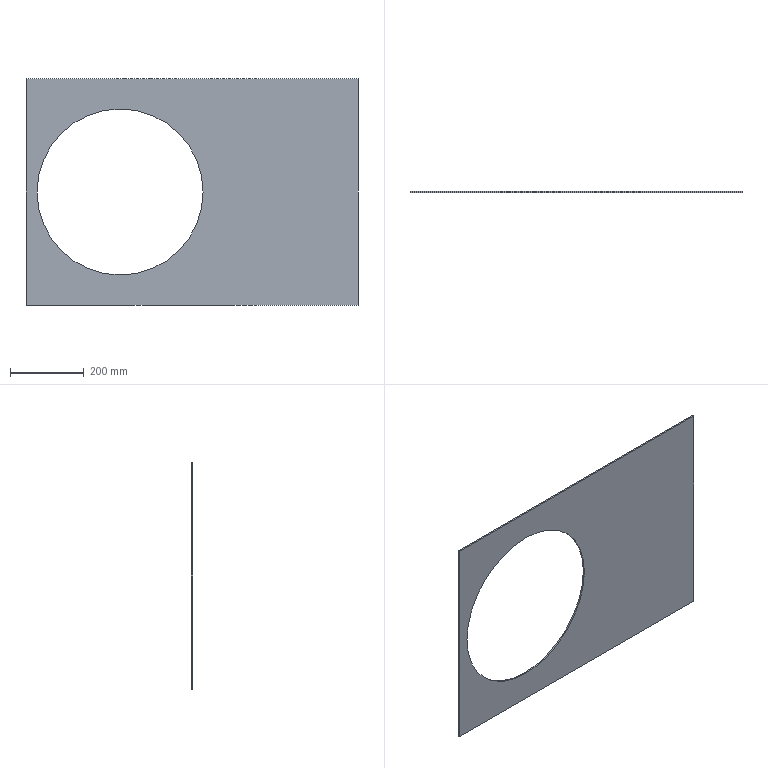Component | SolidWorks | Panel-1 | 1 solid | 8 faces | box 900 x 4 x 615 mm | volume 1577827 mm3 | plane 6 | cylinder 2 | commonest cylinder face diameters 450 x2
build123d program:
from build123d import *

# Parameters (mm, degrees)
SKETCH1_W      = 900
SKETCH1_H      = 615
SKETCH1_R      = 225
EXTRUDE1_DEPTH = 4


with BuildPart() as part:
    # Sketch1 → Extrude1 (new body)
    with BuildSketch(Plane(origin=(0, 0, 0), x_dir=(1, 0, 0), z_dir=(0, 1, 0))):
        with Locations((392.086, -275.962)):
            Rectangle(SKETCH1_W, SKETCH1_H)
        with Locations(Location((197.086, -275.962, 0), (0, 0, 270))):
            Circle(SKETCH1_R, mode=Mode.SUBTRACT)
    extrude(amount=EXTRUDE1_DEPTH)


solid = part.part

# Placed as in the assembly
solid = solid.moved(Location((-361.87, 366.983, -271.962), (0, 0, 0)))
STEP:
#1=CARTESIAN_POINT('',(-6.488,14.606,-8.701));
#2=VERTEX_POINT('',#1);
#3=CARTESIAN_POINT('',(-6.488,14.606,9.016));
#4=VERTEX_POINT('',#3);
#5=CARTESIAN_POINT('',(-6.488,14.606,0.1575));
#6=DIRECTION('',(0.,1.,0.));
#7=DIRECTION('',(0.,0.,1.));
#8=AXIS2_PLACEMENT_3D('',#5,#6,#7);
#9=CIRCLE('',#8,8.858);
#10=EDGE_CURVE('',#2,#4,#9,.T.);
#11=ORIENTED_EDGE('',*,*,#10,.T.);
#12=CARTESIAN_POINT('',(-6.488,14.448,9.016));
#13=VERTEX_POINT('',#12);
#14=CARTESIAN_POINT('',(-6.488,14.606,9.016));
#15=DIRECTION('',(0.,-1.,0.));
#16=VECTOR('',#15,39.37);
#17=LINE('',#14,#16);
#18=EDGE_CURVE('',#4,#13,#17,.T.);
#19=ORIENTED_EDGE('',*,*,#18,.T.);
#20=CARTESIAN_POINT('',(-6.488,14.448,-8.701));
#21=VERTEX_POINT('',#20);
#22=CARTESIAN_POINT('',(-6.488,14.448,0.1575));
#23=DIRECTION('',(0.,1.,0.));
#24=DIRECTION('',(0.,0.,1.));
#25=AXIS2_PLACEMENT_3D('',#22,#23,#24);
#26=CIRCLE('',#25,8.858);
#27=EDGE_CURVE('',#21,#13,#26,.T.);
#28=ORIENTED_EDGE('',*,*,#27,.F.);
#29=CARTESIAN_POINT('',(-6.488,14.606,-8.701));
#30=DIRECTION('',(0.,-1.,0.));
#31=VECTOR('',#30,39.37);
#32=LINE('',#29,#31);
#33=EDGE_CURVE('',#2,#21,#32,.T.);
#34=ORIENTED_EDGE('',*,*,#33,.F.);
#35=EDGE_LOOP('',(#11,#19,#28,#34));
#36=FACE_OUTER_BOUND('',#35,.T.);
#37=CARTESIAN_POINT('',(-6.488,14.606,0.1575));
#38=DIRECTION('',(0.,-1.,0.));
#39=DIRECTION('',(0.,0.,-1.));
#40=AXIS2_PLACEMENT_3D('',#37,#38,#39);
#41=CYLINDRICAL_SURFACE('',#40,8.858);
#42=ADVANCED_FACE('',(#36),#41,.F.);
#43=CARTESIAN_POINT('',(-16.527,14.606,-11.949));
#44=VERTEX_POINT('',#43);
#45=CARTESIAN_POINT('',(-16.527,14.606,12.264));
#46=VERTEX_POINT('',#45);
#47=CARTESIAN_POINT('',(-16.527,14.606,-11.949));
#48=DIRECTION('',(-0.,0.,1.));
#49=VECTOR('',#48,39.37);
#50=LINE('',#47,#49);
#51=EDGE_CURVE('',#44,#46,#50,.T.);
#52=ORIENTED_EDGE('',*,*,#51,.T.);
#53=CARTESIAN_POINT('',(18.906,14.606,12.264));
#54=VERTEX_POINT('',#53);
#55=CARTESIAN_POINT('',(-16.527,14.606,12.264));
#56=DIRECTION('',(1.,0.,0.));
#57=VECTOR('',#56,39.37);
#58=LINE('',#55,#57);
#59=EDGE_CURVE('',#46,#54,#58,.T.);
#60=ORIENTED_EDGE('',*,*,#59,.T.);
#61=CARTESIAN_POINT('',(18.906,14.606,-11.949));
#62=VERTEX_POINT('',#61);
#63=CARTESIAN_POINT('',(18.906,14.606,-11.949));
#64=DIRECTION('',(-0.,0.,-1.));
#65=VECTOR('',#64,39.37);
#66=LINE('',#63,#65);
#67=EDGE_CURVE('',#54,#62,#66,.T.);
#68=ORIENTED_EDGE('',*,*,#67,.T.);
#69=CARTESIAN_POINT('',(-16.527,14.606,-11.949));
#70=DIRECTION('',(-1.,0.,-0.));
#71=VECTOR('',#70,39.37);
#72=LINE('',#69,#71);
#73=EDGE_CURVE('',#62,#44,#72,.T.);
#74=ORIENTED_EDGE('',*,*,#73,.T.);
#75=EDGE_LOOP('',(#52,#60,#68,#74));
#76=FACE_OUTER_BOUND('',#75,.T.);
#77=ORIENTED_EDGE('',*,*,#10,.F.);
#78=CARTESIAN_POINT('',(-6.488,14.606,0.1575));
#79=DIRECTION('',(0.,1.,0.));
#80=DIRECTION('',(0.,0.,1.));
#81=AXIS2_PLACEMENT_3D('',#78,#79,#80);
#82=CIRCLE('',#81,8.858);
#83=EDGE_CURVE('',#4,#2,#82,.T.);
#84=ORIENTED_EDGE('',*,*,#83,.F.);
#85=EDGE_LOOP('',(#77,#84));
#86=FACE_BOUND('',#85,.T.);
#87=CARTESIAN_POINT('',(-16.527,14.606,12.264));
#88=DIRECTION('',(0.,1.,0.));
#89=DIRECTION('',(0.,0.,1.));
#90=AXIS2_PLACEMENT_3D('',#87,#88,#89);
#91=PLANE('',#90);
#92=ADVANCED_FACE('',(#76,#86),#91,.T.);
#93=CARTESIAN_POINT('',(-16.527,14.448,-11.949));
#94=VERTEX_POINT('',#93);
#95=CARTESIAN_POINT('',(-16.527,14.448,12.264));
#96=VERTEX_POINT('',#95);
#97=CARTESIAN_POINT('',(-16.527,14.448,-11.949));
#98=DIRECTION('',(-0.,0.,1.));
#99=VECTOR('',#98,39.37);
#100=LINE('',#97,#99);
#101=EDGE_CURVE('',#94,#96,#100,.T.);
#102=ORIENTED_EDGE('',*,*,#101,.F.);
#103=CARTESIAN_POINT('',(18.906,14.448,-11.949));
#104=VERTEX_POINT('',#103);
#105=CARTESIAN_POINT('',(-16.527,14.448,-11.949));
#106=DIRECTION('',(-1.,0.,-0.));
#107=VECTOR('',#106,39.37);
#108=LINE('',#105,#107);
#109=EDGE_CURVE('',#104,#94,#108,.T.);
#110=ORIENTED_EDGE('',*,*,#109,.F.);
#111=CARTESIAN_POINT('',(18.906,14.448,12.264));
#112=VERTEX_POINT('',#111);
#113=CARTESIAN_POINT('',(18.906,14.448,-11.949));
#114=DIRECTION('',(-0.,0.,-1.));
#115=VECTOR('',#114,39.37);
#116=LINE('',#113,#115);
#117=EDGE_CURVE('',#112,#104,#116,.T.);
#118=ORIENTED_EDGE('',*,*,#117,.F.);
#119=CARTESIAN_POINT('',(-16.527,14.448,12.264));
#120=DIRECTION('',(1.,0.,0.));
#121=VECTOR('',#120,39.37);
#122=LINE('',#119,#121);
#123=EDGE_CURVE('',#96,#112,#122,.T.);
#124=ORIENTED_EDGE('',*,*,#123,.F.);
#125=EDGE_LOOP('',(#102,#110,#118,#124));
#126=FACE_OUTER_BOUND('',#125,.T.);
#127=ORIENTED_EDGE('',*,*,#27,.T.);
#128=CARTESIAN_POINT('',(-6.488,14.448,0.1575));
#129=DIRECTION('',(0.,1.,0.));
#130=DIRECTION('',(0.,0.,1.));
#131=AXIS2_PLACEMENT_3D('',#128,#129,#130);
#132=CIRCLE('',#131,8.858);
#133=EDGE_CURVE('',#13,#21,#132,.T.);
#134=ORIENTED_EDGE('',*,*,#133,.T.);
#135=EDGE_LOOP('',(#127,#134));
#136=FACE_BOUND('',#135,.T.);
#137=CARTESIAN_POINT('',(-16.527,14.448,12.264));
#138=DIRECTION('',(0.,1.,0.));
#139=DIRECTION('',(0.,0.,1.));
#140=AXIS2_PLACEMENT_3D('',#137,#138,#139);
#141=PLANE('',#140);
#142=ADVANCED_FACE('',(#126,#136),#141,.F.);
#143=ORIENTED_EDGE('',*,*,#101,.T.);
#144=CARTESIAN_POINT('',(-16.527,14.606,12.264));
#145=DIRECTION('',(0.,-1.,0.));
#146=VECTOR('',#145,39.37);
#147=LINE('',#144,#146);
#148=EDGE_CURVE('',#46,#96,#147,.T.);
#149=ORIENTED_EDGE('',*,*,#148,.F.);
#150=ORIENTED_EDGE('',*,*,#51,.F.);
#151=CARTESIAN_POINT('',(-16.527,14.606,-11.949));
#152=DIRECTION('',(0.,-1.,0.));
#153=VECTOR('',#152,39.37);
#154=LINE('',#151,#153);
#155=EDGE_CURVE('',#44,#94,#154,.T.);
#156=ORIENTED_EDGE('',*,*,#155,.T.);
#157=EDGE_LOOP('',(#143,#149,#150,#156));
#158=FACE_OUTER_BOUND('',#157,.T.);
#159=CARTESIAN_POINT('',(-16.527,14.606,-11.949));
#160=DIRECTION('',(1.,0.,0.));
#161=DIRECTION('',(0.,0.,-1.));
#162=AXIS2_PLACEMENT_3D('',#159,#160,#161);
#163=PLANE('',#162);
#164=ADVANCED_FACE('',(#158),#163,.F.);
#165=ORIENTED_EDGE('',*,*,#123,.T.);
#166=CARTESIAN_POINT('',(18.906,14.606,12.264));
#167=DIRECTION('',(0.,-1.,0.));
#168=VECTOR('',#167,39.37);
#169=LINE('',#166,#168);
#170=EDGE_CURVE('',#54,#112,#169,.T.);
#171=ORIENTED_EDGE('',*,*,#170,.F.);
#172=ORIENTED_EDGE('',*,*,#59,.F.);
#173=ORIENTED_EDGE('',*,*,#148,.T.);
#174=EDGE_LOOP('',(#165,#171,#172,#173));
#175=FACE_OUTER_BOUND('',#174,.T.);
#176=CARTESIAN_POINT('',(-16.527,14.606,12.264));
#177=DIRECTION('',(0.,0.,-1.));
#178=DIRECTION('',(-1.,0.,0.));
#179=AXIS2_PLACEMENT_3D('',#176,#177,#178);
#180=PLANE('',#179);
#181=ADVANCED_FACE('',(#175),#180,.F.);
#182=ORIENTED_EDGE('',*,*,#117,.T.);
#183=CARTESIAN_POINT('',(18.906,14.606,-11.949));
#184=DIRECTION('',(0.,-1.,0.));
#185=VECTOR('',#184,39.37);
#186=LINE('',#183,#185);
#187=EDGE_CURVE('',#62,#104,#186,.T.);
#188=ORIENTED_EDGE('',*,*,#187,.F.);
#189=ORIENTED_EDGE('',*,*,#67,.F.);
#190=ORIENTED_EDGE('',*,*,#170,.T.);
#191=EDGE_LOOP('',(#182,#188,#189,#190));
#192=FACE_OUTER_BOUND('',#191,.T.);
#193=CARTESIAN_POINT('',(18.906,14.606,-11.949));
#194=DIRECTION('',(-1.,0.,0.));
#195=DIRECTION('',(0.,0.,1.));
#196=AXIS2_PLACEMENT_3D('',#193,#194,#195);
#197=PLANE('',#196);
#198=ADVANCED_FACE('',(#192),#197,.F.);
#199=ORIENTED_EDGE('',*,*,#109,.T.);
#200=ORIENTED_EDGE('',*,*,#155,.F.);
#201=ORIENTED_EDGE('',*,*,#73,.F.);
#202=ORIENTED_EDGE('',*,*,#187,.T.);
#203=EDGE_LOOP('',(#199,#200,#201,#202));
#204=FACE_OUTER_BOUND('',#203,.T.);
#205=CARTESIAN_POINT('',(-16.527,14.606,-11.949));
#206=DIRECTION('',(-0.,0.,1.));
#207=DIRECTION('',(1.,0.,0.));
#208=AXIS2_PLACEMENT_3D('',#205,#206,#207);
#209=PLANE('',#208);
#210=ADVANCED_FACE('',(#204),#209,.F.);
#211=ORIENTED_EDGE('',*,*,#18,.F.);
#212=ORIENTED_EDGE('',*,*,#83,.T.);
#213=ORIENTED_EDGE('',*,*,#33,.T.);
#214=ORIENTED_EDGE('',*,*,#133,.F.);
#215=EDGE_LOOP('',(#211,#212,#213,#214));
#216=FACE_OUTER_BOUND('',#215,.T.);
#217=CARTESIAN_POINT('',(-6.488,14.606,0.1575));
#218=DIRECTION('',(0.,-1.,0.));
#219=DIRECTION('',(0.,0.,-1.));
#220=AXIS2_PLACEMENT_3D('',#217,#218,#219);
#221=CYLINDRICAL_SURFACE('',#220,8.858);
#222=ADVANCED_FACE('',(#216),#221,.F.);
#223=CLOSED_SHELL('',(#42,#92,#142,#164,#181,#198,#210,#222));
#224=MANIFOLD_SOLID_BREP('',#223);
#225=CARTESIAN_POINT('',(0.,0.,0.));
#226=DIRECTION('',(0.,0.,1.));
#227=DIRECTION('',(1.,0.,0.));
#228=AXIS2_PLACEMENT_3D('',#225,#226,#227);
#229=(LENGTH_UNIT()NAMED_UNIT(*)SI_UNIT($,.METRE.));
#230=LENGTH_MEASURE_WITH_UNIT(LENGTH_MEASURE(0.0254),#229);
#231=DIMENSIONAL_EXPONENTS(1.,0.,0.,0.,0.,0.,0.);
#232=(CONVERSION_BASED_UNIT('',#230)LENGTH_UNIT()NAMED_UNIT(#231));
#233=UNCERTAINTY_MEASURE_WITH_UNIT(LENGTH_MEASURE(0.00001),#232,'','');
#234=(NAMED_UNIT(*)PLANE_ANGLE_UNIT()SI_UNIT($,.RADIAN.));
#235=(NAMED_UNIT(*)SI_UNIT($,.STERADIAN.)SOLID_ANGLE_UNIT());
#236=(GEOMETRIC_REPRESENTATION_CONTEXT(3)GLOBAL_UNCERTAINTY_ASSIGNED_CONTEXT((#233))GLOBAL_UNIT_ASSIGNED_CONTEXT((#232,#234,#235))REPRESENTATION_CONTEXT('',''));
#237=ADVANCED_BREP_SHAPE_REPRESENTATION('',(#224,#228),#236);
#238=COLOUR_RGB('',0.7922,0.8196,0.9333);
#239=FILL_AREA_STYLE_COLOUR('',#238);
#240=FILL_AREA_STYLE('',(#239));
#241=SURFACE_STYLE_FILL_AREA(#240);
#242=SURFACE_SIDE_STYLE('',(#241));
#243=SURFACE_STYLE_USAGE(.BOTH.,#242);
#244=PRESENTATION_STYLE_ASSIGNMENT((#243));
#245=STYLED_ITEM('',(#244),#224);
#246=(LENGTH_UNIT()NAMED_UNIT(*)SI_UNIT($,.METRE.));
#247=LENGTH_MEASURE_WITH_UNIT(LENGTH_MEASURE(0.0254),#246);
#248=DIMENSIONAL_EXPONENTS(1.,0.,0.,0.,0.,0.,0.);
#249=(CONVERSION_BASED_UNIT('',#247)LENGTH_UNIT()NAMED_UNIT(#248));
#250=UNCERTAINTY_MEASURE_WITH_UNIT(LENGTH_MEASURE(0.00001),#249,'','');
#251=(NAMED_UNIT(*)PLANE_ANGLE_UNIT()SI_UNIT($,.RADIAN.));
#252=(NAMED_UNIT(*)SI_UNIT($,.STERADIAN.)SOLID_ANGLE_UNIT());
#253=(GEOMETRIC_REPRESENTATION_CONTEXT(3)GLOBAL_UNCERTAINTY_ASSIGNED_CONTEXT((#250))GLOBAL_UNIT_ASSIGNED_CONTEXT((#249,#251,#252))REPRESENTATION_CONTEXT('',''));
#254=MECHANICAL_DESIGN_GEOMETRIC_PRESENTATION_REPRESENTATION('',(#245),#253);
#255=PRESENTATION_LAYER_ASSIGNMENT('','',(#245));